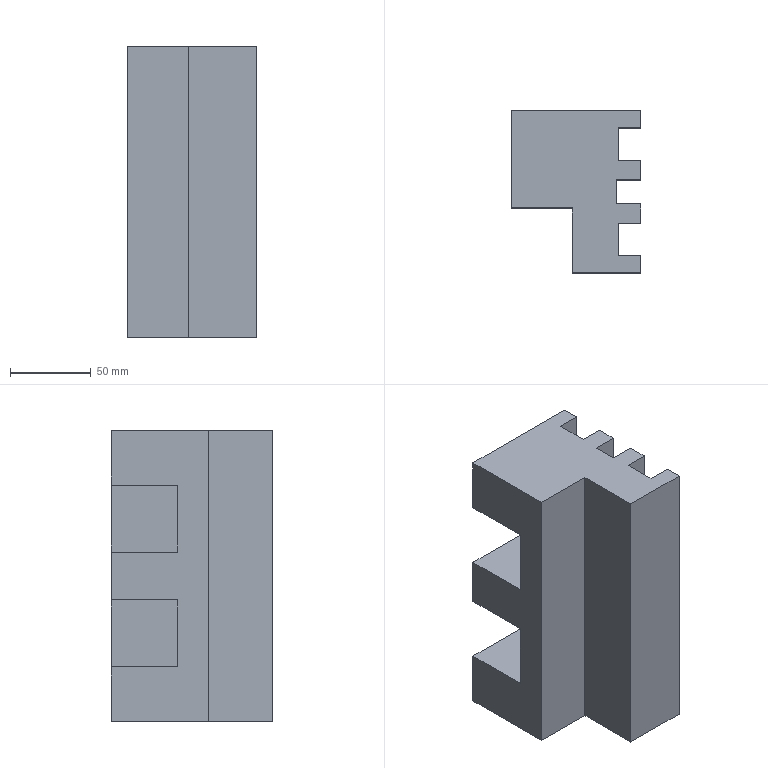Component | SolidWorks | Fixture-2 | 1 solid | 28 faces | box 80 x 100 x 180 mm | volume 866480 mm3 | plane 28
build123d program:
from build123d import *

# Parameters (mm, degrees)
BOSS_EXTRUDE1_DEPTH     = 180
SKETCH2_W               = 46.727
SKETCH2_H               = 41.35
CUT_EXTRUDE1_DEPTH      = 30
CUT_EXTRUDE2_DEPTH      = 221.907
CUT_EXTRUDE2_DEPTH_BACK = 221.907
SKETCH3_W               = 15
SKETCH3_H               = 15
CUT_EXTRUDE3_DEPTH      = 221.907
CUT_EXTRUDE3_DEPTH_BACK = 221.907
SKETCH4_W               = 14
SKETCH4_H               = 20
SKETCH5_W               = 46.727
SKETCH5_H               = 41.35
CUT_EXTRUDE4_DEPTH      = 11.35


with BuildPart() as part:
    # Sketch1 → Boss-Extrude1 (new body)
    with BuildSketch(Plane.XY):
        Polygon((0, 0), (-80, 0), (-80, -60), (-42.162, -60), (-42.162, -100), (0, -100), align=None)
    extrude(amount=BOSS_EXTRUDE1_DEPTH)

    # Sketch2 → Cut-Extrude1 (cut)
    with BuildSketch(Plane(origin=(0, 0, 0), x_dir=(1, 0, 0), z_dir=(0, 1, 0))):
        with Locations((-56.637, -125.435)):
            Rectangle(SKETCH2_W, SKETCH2_H)
        with Locations((-56.637, -54.565)):
            Rectangle(SKETCH2_W, SKETCH2_H)
    extrude(amount=-CUT_EXTRUDE1_DEPTH, mode=Mode.SUBTRACT)

    # Sketch3 → Cut-Extrude2 (cut, two sides: drawn at the far end of the back side and taken through both)
    with BuildSketch(Plane(origin=(0, 0, 0), x_dir=(-1, 0, 0), z_dir=(0, 0, -1)).offset(-CUT_EXTRUDE2_DEPTH_BACK)):
        with Locations((7.5, -50)):
            Rectangle(SKETCH3_W, SKETCH3_H)
    extrude(amount=CUT_EXTRUDE2_DEPTH + CUT_EXTRUDE2_DEPTH_BACK, mode=Mode.SUBTRACT)

    # Sketch4 → Cut-Extrude3 (cut, two sides: drawn at the far end of the back side and taken through both)
    with BuildSketch(Plane(origin=(0, 0, 0), x_dir=(-1, 0, 0), z_dir=(0, 0, -1)).offset(-CUT_EXTRUDE3_DEPTH_BACK)):
        with Locations((7, -20.5)):
            Rectangle(SKETCH4_W, SKETCH4_H)
        with Locations((7, -79.5)):
            Rectangle(SKETCH4_W, SKETCH4_H)
    extrude(amount=CUT_EXTRUDE3_DEPTH + CUT_EXTRUDE3_DEPTH_BACK, mode=Mode.SUBTRACT)

    # Sketch5 → Cut-Extrude4 (cut)
    with BuildSketch(Plane(origin=(0, -30, 0), x_dir=(1, 0, 0), z_dir=(0, 1, 0))):
        with Locations((-56.637, -125.435)):
            Rectangle(SKETCH5_W, SKETCH5_H)
        with Locations((-56.637, -54.565)):
            Rectangle(SKETCH5_W, SKETCH5_H)
    extrude(amount=-CUT_EXTRUDE4_DEPTH, mode=Mode.SUBTRACT)


solid = part.part

# Placed as in the assembly
solid = solid.moved(Location((-136.557, 55.832, -117.351), (0, 0, 0)))
STEP:
#1=COLOUR_RGB('',0.7922,0.8196,0.9333);
#2=FILL_AREA_STYLE_COLOUR('',#1);
#3=FILL_AREA_STYLE('',(#2));
#4=SURFACE_STYLE_FILL_AREA(#3);
#5=SURFACE_SIDE_STYLE('',(#4));
#6=SURFACE_STYLE_USAGE(.BOTH.,#5);
#7=PRESENTATION_STYLE_ASSIGNMENT((#6));
#8=CARTESIAN_POINT('',(-5.376,1.785,2.466));
#9=VERTEX_POINT('',#8);
#10=CARTESIAN_POINT('',(-5.376,2.198,2.466));
#11=VERTEX_POINT('',#10);
#12=CARTESIAN_POINT('',(-5.376,2.198,2.466));
#13=DIRECTION('',(-0.,1.,0.));
#14=VECTOR('',#13,39.37);
#15=LINE('',#12,#14);
#16=EDGE_CURVE('',#9,#11,#15,.T.);
#17=ORIENTED_EDGE('',*,*,#16,.F.);
#18=CARTESIAN_POINT('',(-5.376,1.785,-4.62));
#19=VERTEX_POINT('',#18);
#20=CARTESIAN_POINT('',(-5.376,1.785,2.466));
#21=DIRECTION('',(0.,0.,-1.));
#22=VECTOR('',#21,39.37);
#23=LINE('',#20,#22);
#24=EDGE_CURVE('',#9,#19,#23,.T.);
#25=ORIENTED_EDGE('',*,*,#24,.T.);
#26=CARTESIAN_POINT('',(-5.376,2.198,-4.62));
#27=VERTEX_POINT('',#26);
#28=CARTESIAN_POINT('',(-5.376,2.198,-4.62));
#29=DIRECTION('',(-0.,1.,0.));
#30=VECTOR('',#29,39.37);
#31=LINE('',#28,#30);
#32=EDGE_CURVE('',#19,#27,#31,.T.);
#33=ORIENTED_EDGE('',*,*,#32,.T.);
#34=CARTESIAN_POINT('',(-5.376,2.198,2.466));
#35=DIRECTION('',(0.,0.,-1.));
#36=VECTOR('',#35,39.37);
#37=LINE('',#34,#36);
#38=EDGE_CURVE('',#11,#27,#37,.T.);
#39=ORIENTED_EDGE('',*,*,#38,.F.);
#40=EDGE_LOOP('',(#17,#25,#33,#39));
#41=FACE_OUTER_BOUND('',#40,.T.);
#42=CARTESIAN_POINT('',(-5.376,2.198,2.466));
#43=DIRECTION('',(-1.,-0.,0.));
#44=DIRECTION('',(0.,-1.,0.));
#45=AXIS2_PLACEMENT_3D('',#42,#43,#44);
#46=PLANE('',#45);
#47=ADVANCED_FACE('',(#41),#46,.F.);
#48=CARTESIAN_POINT('',(-5.376,-1.739,-4.62));
#49=VERTEX_POINT('',#48);
#50=CARTESIAN_POINT('',(-5.376,-1.326,-4.62));
#51=VERTEX_POINT('',#50);
#52=CARTESIAN_POINT('',(-5.376,2.198,-4.62));
#53=DIRECTION('',(-0.,1.,0.));
#54=VECTOR('',#53,39.37);
#55=LINE('',#52,#54);
#56=EDGE_CURVE('',#49,#51,#55,.T.);
#57=ORIENTED_EDGE('',*,*,#56,.T.);
#58=CARTESIAN_POINT('',(-5.376,-1.326,2.466));
#59=VERTEX_POINT('',#58);
#60=CARTESIAN_POINT('',(-5.376,-1.326,2.466));
#61=DIRECTION('',(0.,0.,-1.));
#62=VECTOR('',#61,39.37);
#63=LINE('',#60,#62);
#64=EDGE_CURVE('',#59,#51,#63,.T.);
#65=ORIENTED_EDGE('',*,*,#64,.F.);
#66=CARTESIAN_POINT('',(-5.376,-1.739,2.466));
#67=VERTEX_POINT('',#66);
#68=CARTESIAN_POINT('',(-5.376,2.198,2.466));
#69=DIRECTION('',(-0.,1.,0.));
#70=VECTOR('',#69,39.37);
#71=LINE('',#68,#70);
#72=EDGE_CURVE('',#67,#59,#71,.T.);
#73=ORIENTED_EDGE('',*,*,#72,.F.);
#74=CARTESIAN_POINT('',(-5.376,-1.739,2.466));
#75=DIRECTION('',(0.,0.,-1.));
#76=VECTOR('',#75,39.37);
#77=LINE('',#74,#76);
#78=EDGE_CURVE('',#67,#49,#77,.T.);
#79=ORIENTED_EDGE('',*,*,#78,.T.);
#80=EDGE_LOOP('',(#57,#65,#73,#79));
#81=FACE_OUTER_BOUND('',#80,.T.);
#82=CARTESIAN_POINT('',(-5.376,2.198,2.466));
#83=DIRECTION('',(-1.,-0.,0.));
#84=DIRECTION('',(0.,-1.,0.));
#85=AXIS2_PLACEMENT_3D('',#82,#83,#84);
#86=PLANE('',#85);
#87=ADVANCED_FACE('',(#81),#86,.F.);
#88=CARTESIAN_POINT('',(-5.376,0.5249,-4.62));
#89=VERTEX_POINT('',#88);
#90=CARTESIAN_POINT('',(-5.376,0.9973,-4.62));
#91=VERTEX_POINT('',#90);
#92=CARTESIAN_POINT('',(-5.376,2.198,-4.62));
#93=DIRECTION('',(-0.,1.,0.));
#94=VECTOR('',#93,39.37);
#95=LINE('',#92,#94);
#96=EDGE_CURVE('',#89,#91,#95,.T.);
#97=ORIENTED_EDGE('',*,*,#96,.T.);
#98=CARTESIAN_POINT('',(-5.376,0.9973,2.466));
#99=VERTEX_POINT('',#98);
#100=CARTESIAN_POINT('',(-5.376,0.9973,2.466));
#101=DIRECTION('',(0.,0.,-1.));
#102=VECTOR('',#101,39.37);
#103=LINE('',#100,#102);
#104=EDGE_CURVE('',#99,#91,#103,.T.);
#105=ORIENTED_EDGE('',*,*,#104,.F.);
#106=CARTESIAN_POINT('',(-5.376,0.5249,2.466));
#107=VERTEX_POINT('',#106);
#108=CARTESIAN_POINT('',(-5.376,2.198,2.466));
#109=DIRECTION('',(-0.,1.,0.));
#110=VECTOR('',#109,39.37);
#111=LINE('',#108,#110);
#112=EDGE_CURVE('',#107,#99,#111,.T.);
#113=ORIENTED_EDGE('',*,*,#112,.F.);
#114=CARTESIAN_POINT('',(-5.376,0.5249,2.466));
#115=DIRECTION('',(0.,0.,-1.));
#116=VECTOR('',#115,39.37);
#117=LINE('',#114,#116);
#118=EDGE_CURVE('',#107,#89,#117,.T.);
#119=ORIENTED_EDGE('',*,*,#118,.T.);
#120=EDGE_LOOP('',(#97,#105,#113,#119));
#121=FACE_OUTER_BOUND('',#120,.T.);
#122=CARTESIAN_POINT('',(-5.376,2.198,2.466));
#123=DIRECTION('',(-1.,-0.,0.));
#124=DIRECTION('',(0.,-1.,0.));
#125=AXIS2_PLACEMENT_3D('',#122,#123,#124);
#126=PLANE('',#125);
#127=ADVANCED_FACE('',(#121),#126,.F.);
#128=CARTESIAN_POINT('',(-8.526,2.198,-0.4957));
#129=VERTEX_POINT('',#128);
#130=CARTESIAN_POINT('',(-6.686,2.198,-0.4957));
#131=VERTEX_POINT('',#130);
#132=CARTESIAN_POINT('',(-5.376,2.198,-0.4957));
#133=DIRECTION('',(1.,0.,0.));
#134=VECTOR('',#133,39.37);
#135=LINE('',#132,#134);
#136=EDGE_CURVE('',#129,#131,#135,.T.);
#137=ORIENTED_EDGE('',*,*,#136,.T.);
#138=CARTESIAN_POINT('',(-6.686,2.198,1.132));
#139=VERTEX_POINT('',#138);
#140=CARTESIAN_POINT('',(-6.686,2.198,-4.62));
#141=DIRECTION('',(0.,0.,-1.));
#142=VECTOR('',#141,39.37);
#143=LINE('',#140,#142);
#144=EDGE_CURVE('',#139,#131,#143,.T.);
#145=ORIENTED_EDGE('',*,*,#144,.F.);
#146=CARTESIAN_POINT('',(-8.526,2.198,1.132));
#147=VERTEX_POINT('',#146);
#148=CARTESIAN_POINT('',(-5.376,2.198,1.132));
#149=DIRECTION('',(1.,0.,0.));
#150=VECTOR('',#149,39.37);
#151=LINE('',#148,#150);
#152=EDGE_CURVE('',#147,#139,#151,.T.);
#153=ORIENTED_EDGE('',*,*,#152,.F.);
#154=CARTESIAN_POINT('',(-8.526,2.198,2.466));
#155=VERTEX_POINT('',#154);
#156=CARTESIAN_POINT('',(-8.526,2.198,2.466));
#157=DIRECTION('',(0.,0.,-1.));
#158=VECTOR('',#157,39.37);
#159=LINE('',#156,#158);
#160=EDGE_CURVE('',#155,#147,#159,.T.);
#161=ORIENTED_EDGE('',*,*,#160,.F.);
#162=CARTESIAN_POINT('',(-5.376,2.198,2.466));
#163=DIRECTION('',(-1.,-0.,0.));
#164=VECTOR('',#163,39.37);
#165=LINE('',#162,#164);
#166=EDGE_CURVE('',#11,#155,#165,.T.);
#167=ORIENTED_EDGE('',*,*,#166,.F.);
#168=ORIENTED_EDGE('',*,*,#38,.T.);
#169=CARTESIAN_POINT('',(-8.526,2.198,-4.62));
#170=VERTEX_POINT('',#169);
#171=CARTESIAN_POINT('',(-5.376,2.198,-4.62));
#172=DIRECTION('',(-1.,-0.,0.));
#173=VECTOR('',#172,39.37);
#174=LINE('',#171,#173);
#175=EDGE_CURVE('',#27,#170,#174,.T.);
#176=ORIENTED_EDGE('',*,*,#175,.T.);
#177=CARTESIAN_POINT('',(-8.526,2.198,-3.286));
#178=VERTEX_POINT('',#177);
#179=CARTESIAN_POINT('',(-8.526,2.198,2.466));
#180=DIRECTION('',(0.,0.,-1.));
#181=VECTOR('',#180,39.37);
#182=LINE('',#179,#181);
#183=EDGE_CURVE('',#178,#170,#182,.T.);
#184=ORIENTED_EDGE('',*,*,#183,.F.);
#185=CARTESIAN_POINT('',(-6.686,2.198,-3.286));
#186=VERTEX_POINT('',#185);
#187=CARTESIAN_POINT('',(-8.526,2.198,-3.286));
#188=DIRECTION('',(1.,0.,0.));
#189=VECTOR('',#188,39.37);
#190=LINE('',#187,#189);
#191=EDGE_CURVE('',#178,#186,#190,.T.);
#192=ORIENTED_EDGE('',*,*,#191,.T.);
#193=CARTESIAN_POINT('',(-6.686,2.198,-1.658));
#194=VERTEX_POINT('',#193);
#195=CARTESIAN_POINT('',(-6.686,2.198,-3.286));
#196=DIRECTION('',(0.,0.,1.));
#197=VECTOR('',#196,39.37);
#198=LINE('',#195,#197);
#199=EDGE_CURVE('',#186,#194,#198,.T.);
#200=ORIENTED_EDGE('',*,*,#199,.T.);
#201=CARTESIAN_POINT('',(-8.526,2.198,-1.658));
#202=VERTEX_POINT('',#201);
#203=CARTESIAN_POINT('',(-8.526,2.198,-1.658));
#204=DIRECTION('',(1.,0.,0.));
#205=VECTOR('',#204,39.37);
#206=LINE('',#203,#205);
#207=EDGE_CURVE('',#202,#194,#206,.T.);
#208=ORIENTED_EDGE('',*,*,#207,.F.);
#209=CARTESIAN_POINT('',(-8.526,2.198,2.466));
#210=DIRECTION('',(0.,0.,-1.));
#211=VECTOR('',#210,39.37);
#212=LINE('',#209,#211);
#213=EDGE_CURVE('',#129,#202,#212,.T.);
#214=ORIENTED_EDGE('',*,*,#213,.F.);
#215=EDGE_LOOP('',(#137,#145,#153,#161,#167,#168,#176,#184,#192,#200,#208,#214));
#216=FACE_OUTER_BOUND('',#215,.T.);
#217=CARTESIAN_POINT('',(-5.376,2.198,2.466));
#218=DIRECTION('',(0.,-1.,0.));
#219=DIRECTION('',(1.,0.,0.));
#220=AXIS2_PLACEMENT_3D('',#217,#218,#219);
#221=PLANE('',#220);
#222=ADVANCED_FACE('',(#216),#221,.F.);
#223=CARTESIAN_POINT('',(-8.526,0.5701,-0.4957));
#224=VERTEX_POINT('',#223);
#225=CARTESIAN_POINT('',(-8.526,0.5701,1.132));
#226=VERTEX_POINT('',#225);
#227=CARTESIAN_POINT('',(-8.526,0.5701,-0.4957));
#228=DIRECTION('',(-0.,0.,1.));
#229=VECTOR('',#228,39.37);
#230=LINE('',#227,#229);
#231=EDGE_CURVE('',#224,#226,#230,.T.);
#232=ORIENTED_EDGE('',*,*,#231,.F.);
#233=CARTESIAN_POINT('',(-8.526,1.017,-0.4957));
#234=DIRECTION('',(-0.,1.,0.));
#235=VECTOR('',#234,39.37);
#236=LINE('',#233,#235);
#237=EDGE_CURVE('',#224,#129,#236,.T.);
#238=ORIENTED_EDGE('',*,*,#237,.T.);
#239=ORIENTED_EDGE('',*,*,#213,.T.);
#240=CARTESIAN_POINT('',(-8.526,0.5701,-1.658));
#241=VERTEX_POINT('',#240);
#242=CARTESIAN_POINT('',(-8.526,1.017,-1.658));
#243=DIRECTION('',(-0.,1.,0.));
#244=VECTOR('',#243,39.37);
#245=LINE('',#242,#244);
#246=EDGE_CURVE('',#241,#202,#245,.T.);
#247=ORIENTED_EDGE('',*,*,#246,.F.);
#248=CARTESIAN_POINT('',(-8.526,0.5701,-3.286));
#249=VERTEX_POINT('',#248);
#250=CARTESIAN_POINT('',(-8.526,0.5701,-3.286));
#251=DIRECTION('',(-0.,0.,1.));
#252=VECTOR('',#251,39.37);
#253=LINE('',#250,#252);
#254=EDGE_CURVE('',#249,#241,#253,.T.);
#255=ORIENTED_EDGE('',*,*,#254,.F.);
#256=CARTESIAN_POINT('',(-8.526,1.017,-3.286));
#257=DIRECTION('',(-0.,1.,0.));
#258=VECTOR('',#257,39.37);
#259=LINE('',#256,#258);
#260=EDGE_CURVE('',#249,#178,#259,.T.);
#261=ORIENTED_EDGE('',*,*,#260,.T.);
#262=ORIENTED_EDGE('',*,*,#183,.T.);
#263=CARTESIAN_POINT('',(-8.526,-0.1641,-4.62));
#264=VERTEX_POINT('',#263);
#265=CARTESIAN_POINT('',(-8.526,2.198,-4.62));
#266=DIRECTION('',(0.,-1.,0.));
#267=VECTOR('',#266,39.37);
#268=LINE('',#265,#267);
#269=EDGE_CURVE('',#170,#264,#268,.T.);
#270=ORIENTED_EDGE('',*,*,#269,.T.);
#271=CARTESIAN_POINT('',(-8.526,-0.1641,2.466));
#272=VERTEX_POINT('',#271);
#273=CARTESIAN_POINT('',(-8.526,-0.1641,2.466));
#274=DIRECTION('',(0.,0.,-1.));
#275=VECTOR('',#274,39.37);
#276=LINE('',#273,#275);
#277=EDGE_CURVE('',#272,#264,#276,.T.);
#278=ORIENTED_EDGE('',*,*,#277,.F.);
#279=CARTESIAN_POINT('',(-8.526,2.198,2.466));
#280=DIRECTION('',(0.,-1.,0.));
#281=VECTOR('',#280,39.37);
#282=LINE('',#279,#281);
#283=EDGE_CURVE('',#155,#272,#282,.T.);
#284=ORIENTED_EDGE('',*,*,#283,.F.);
#285=ORIENTED_EDGE('',*,*,#160,.T.);
#286=CARTESIAN_POINT('',(-8.526,1.017,1.132));
#287=DIRECTION('',(-0.,1.,0.));
#288=VECTOR('',#287,39.37);
#289=LINE('',#286,#288);
#290=EDGE_CURVE('',#226,#147,#289,.T.);
#291=ORIENTED_EDGE('',*,*,#290,.F.);
#292=EDGE_LOOP('',(#232,#238,#239,#247,#255,#261,#262,#270,#278,#284,#285,#291));
#293=FACE_OUTER_BOUND('',#292,.T.);
#294=CARTESIAN_POINT('',(-8.526,2.198,2.466));
#295=DIRECTION('',(1.,0.,0.));
#296=DIRECTION('',(-0.,1.,0.));
#297=AXIS2_PLACEMENT_3D('',#294,#295,#296);
#298=PLANE('',#297);
#299=ADVANCED_FACE('',(#293),#298,.F.);
#300=CARTESIAN_POINT('',(-5.376,-0.5381,2.466));
#301=VERTEX_POINT('',#300);
#302=CARTESIAN_POINT('',(-5.376,-0.06568,2.466));
#303=VERTEX_POINT('',#302);
#304=CARTESIAN_POINT('',(-5.376,2.198,2.466));
#305=DIRECTION('',(-0.,1.,0.));
#306=VECTOR('',#305,39.37);
#307=LINE('',#304,#306);
#308=EDGE_CURVE('',#301,#303,#307,.T.);
#309=ORIENTED_EDGE('',*,*,#308,.F.);
#310=CARTESIAN_POINT('',(-5.376,-0.5381,-4.62));
#311=VERTEX_POINT('',#310);
#312=CARTESIAN_POINT('',(-5.376,-0.5381,2.466));
#313=DIRECTION('',(0.,0.,-1.));
#314=VECTOR('',#313,39.37);
#315=LINE('',#312,#314);
#316=EDGE_CURVE('',#301,#311,#315,.T.);
#317=ORIENTED_EDGE('',*,*,#316,.T.);
#318=CARTESIAN_POINT('',(-5.376,-0.06568,-4.62));
#319=VERTEX_POINT('',#318);
#320=CARTESIAN_POINT('',(-5.376,2.198,-4.62));
#321=DIRECTION('',(-0.,1.,0.));
#322=VECTOR('',#321,39.37);
#323=LINE('',#320,#322);
#324=EDGE_CURVE('',#311,#319,#323,.T.);
#325=ORIENTED_EDGE('',*,*,#324,.T.);
#326=CARTESIAN_POINT('',(-5.376,-0.06568,2.466));
#327=DIRECTION('',(0.,0.,-1.));
#328=VECTOR('',#327,39.37);
#329=LINE('',#326,#328);
#330=EDGE_CURVE('',#303,#319,#329,.T.);
#331=ORIENTED_EDGE('',*,*,#330,.F.);
#332=EDGE_LOOP('',(#309,#317,#325,#331));
#333=FACE_OUTER_BOUND('',#332,.T.);
#334=CARTESIAN_POINT('',(-5.376,2.198,2.466));
#335=DIRECTION('',(-1.,-0.,0.));
#336=DIRECTION('',(0.,-1.,0.));
#337=AXIS2_PLACEMENT_3D('',#334,#335,#336);
#338=PLANE('',#337);
#339=ADVANCED_FACE('',(#333),#338,.F.);
#340=CARTESIAN_POINT('',(-7.036,-0.1641,-4.62));
#341=VERTEX_POINT('',#340);
#342=CARTESIAN_POINT('',(-7.036,-0.1641,-4.62));
#343=DIRECTION('',(1.,0.,0.));
#344=VECTOR('',#343,39.37);
#345=LINE('',#342,#344);
#346=EDGE_CURVE('',#264,#341,#345,.T.);
#347=ORIENTED_EDGE('',*,*,#346,.T.);
#348=CARTESIAN_POINT('',(-7.036,-0.1641,2.466));
#349=VERTEX_POINT('',#348);
#350=CARTESIAN_POINT('',(-7.036,-0.1641,2.466));
#351=DIRECTION('',(0.,0.,-1.));
#352=VECTOR('',#351,39.37);
#353=LINE('',#350,#352);
#354=EDGE_CURVE('',#349,#341,#353,.T.);
#355=ORIENTED_EDGE('',*,*,#354,.F.);
#356=CARTESIAN_POINT('',(-7.036,-0.1641,2.466));
#357=DIRECTION('',(1.,0.,0.));
#358=VECTOR('',#357,39.37);
#359=LINE('',#356,#358);
#360=EDGE_CURVE('',#272,#349,#359,.T.);
#361=ORIENTED_EDGE('',*,*,#360,.F.);
#362=ORIENTED_EDGE('',*,*,#277,.T.);
#363=EDGE_LOOP('',(#347,#355,#361,#362));
#364=FACE_OUTER_BOUND('',#363,.T.);
#365=CARTESIAN_POINT('',(-7.036,-0.1641,2.466));
#366=DIRECTION('',(-0.,1.,0.));
#367=DIRECTION('',(-1.,-0.,0.));
#368=AXIS2_PLACEMENT_3D('',#365,#366,#367);
#369=PLANE('',#368);
#370=ADVANCED_FACE('',(#364),#369,.F.);
#371=CARTESIAN_POINT('',(-7.036,-1.739,-4.62));
#372=VERTEX_POINT('',#371);
#373=CARTESIAN_POINT('',(-7.036,-1.739,-4.62));
#374=DIRECTION('',(-0.,-1.,0.));
#375=VECTOR('',#374,39.37);
#376=LINE('',#373,#375);
#377=EDGE_CURVE('',#341,#372,#376,.T.);
#378=ORIENTED_EDGE('',*,*,#377,.T.);
#379=CARTESIAN_POINT('',(-7.036,-1.739,2.466));
#380=VERTEX_POINT('',#379);
#381=CARTESIAN_POINT('',(-7.036,-1.739,2.466));
#382=DIRECTION('',(0.,0.,-1.));
#383=VECTOR('',#382,39.37);
#384=LINE('',#381,#383);
#385=EDGE_CURVE('',#380,#372,#384,.T.);
#386=ORIENTED_EDGE('',*,*,#385,.F.);
#387=CARTESIAN_POINT('',(-7.036,-1.739,2.466));
#388=DIRECTION('',(-0.,-1.,0.));
#389=VECTOR('',#388,39.37);
#390=LINE('',#387,#389);
#391=EDGE_CURVE('',#349,#380,#390,.T.);
#392=ORIENTED_EDGE('',*,*,#391,.F.);
#393=ORIENTED_EDGE('',*,*,#354,.T.);
#394=EDGE_LOOP('',(#378,#386,#392,#393));
#395=FACE_OUTER_BOUND('',#394,.T.);
#396=CARTESIAN_POINT('',(-7.036,-1.739,2.466));
#397=DIRECTION('',(1.,-0.,0.));
#398=DIRECTION('',(0.,1.,0.));
#399=AXIS2_PLACEMENT_3D('',#396,#397,#398);
#400=PLANE('',#399);
#401=ADVANCED_FACE('',(#395),#400,.F.);
#402=CARTESIAN_POINT('',(-5.376,-1.739,-4.62));
#403=DIRECTION('',(1.,0.,0.));
#404=VECTOR('',#403,39.37);
#405=LINE('',#402,#404);
#406=EDGE_CURVE('',#372,#49,#405,.T.);
#407=ORIENTED_EDGE('',*,*,#406,.T.);
#408=ORIENTED_EDGE('',*,*,#78,.F.);
#409=CARTESIAN_POINT('',(-5.376,-1.739,2.466));
#410=DIRECTION('',(1.,0.,0.));
#411=VECTOR('',#410,39.37);
#412=LINE('',#409,#411);
#413=EDGE_CURVE('',#380,#67,#412,.T.);
#414=ORIENTED_EDGE('',*,*,#413,.F.);
#415=ORIENTED_EDGE('',*,*,#385,.T.);
#416=EDGE_LOOP('',(#407,#408,#414,#415));
#417=FACE_OUTER_BOUND('',#416,.T.);
#418=CARTESIAN_POINT('',(-5.376,-1.739,2.466));
#419=DIRECTION('',(0.,1.,0.));
#420=DIRECTION('',(0.,0.,1.));
#421=AXIS2_PLACEMENT_3D('',#418,#419,#420);
#422=PLANE('',#421);
#423=ADVANCED_FACE('',(#417),#422,.F.);
#424=CARTESIAN_POINT('',(-5.927,0.9973,2.466));
#425=VERTEX_POINT('',#424);
#426=CARTESIAN_POINT('',(-5.927,1.785,2.466));
#427=VERTEX_POINT('',#426);
#428=CARTESIAN_POINT('',(-5.927,1.785,2.466));
#429=DIRECTION('',(0.,1.,0.));
#430=VECTOR('',#429,39.37);
#431=LINE('',#428,#430);
#432=EDGE_CURVE('',#425,#427,#431,.T.);
#433=ORIENTED_EDGE('',*,*,#432,.T.);
#434=CARTESIAN_POINT('',(-5.376,1.785,2.466));
#435=DIRECTION('',(1.,0.,0.));
#436=VECTOR('',#435,39.37);
#437=LINE('',#434,#436);
#438=EDGE_CURVE('',#427,#9,#437,.T.);
#439=ORIENTED_EDGE('',*,*,#438,.T.);
#440=ORIENTED_EDGE('',*,*,#16,.T.);
#441=ORIENTED_EDGE('',*,*,#166,.T.);
#442=ORIENTED_EDGE('',*,*,#283,.T.);
#443=ORIENTED_EDGE('',*,*,#360,.T.);
#444=ORIENTED_EDGE('',*,*,#391,.T.);
#445=ORIENTED_EDGE('',*,*,#413,.T.);
#446=ORIENTED_EDGE('',*,*,#72,.T.);
#447=CARTESIAN_POINT('',(-5.927,-1.326,2.466));
#448=VERTEX_POINT('',#447);
#449=CARTESIAN_POINT('',(-5.376,-1.326,2.466));
#450=DIRECTION('',(-1.,0.,0.));
#451=VECTOR('',#450,39.37);
#452=LINE('',#449,#451);
#453=EDGE_CURVE('',#59,#448,#452,.T.);
#454=ORIENTED_EDGE('',*,*,#453,.T.);
#455=CARTESIAN_POINT('',(-5.927,-0.5381,2.466));
#456=VERTEX_POINT('',#455);
#457=CARTESIAN_POINT('',(-5.927,-1.326,2.466));
#458=DIRECTION('',(-0.,1.,0.));
#459=VECTOR('',#458,39.37);
#460=LINE('',#457,#459);
#461=EDGE_CURVE('',#448,#456,#460,.T.);
#462=ORIENTED_EDGE('',*,*,#461,.T.);
#463=CARTESIAN_POINT('',(-5.376,-0.5381,2.466));
#464=DIRECTION('',(1.,0.,0.));
#465=VECTOR('',#464,39.37);
#466=LINE('',#463,#465);
#467=EDGE_CURVE('',#456,#301,#466,.T.);
#468=ORIENTED_EDGE('',*,*,#467,.T.);
#469=ORIENTED_EDGE('',*,*,#308,.T.);
#470=CARTESIAN_POINT('',(-5.967,-0.06568,2.466));
#471=VERTEX_POINT('',#470);
#472=CARTESIAN_POINT('',(-5.376,-0.06568,2.466));
#473=DIRECTION('',(-1.,0.,0.));
#474=VECTOR('',#473,39.37);
#475=LINE('',#472,#474);
#476=EDGE_CURVE('',#303,#471,#475,.T.);
#477=ORIENTED_EDGE('',*,*,#476,.T.);
#478=CARTESIAN_POINT('',(-5.967,0.5249,2.466));
#479=VERTEX_POINT('',#478);
#480=CARTESIAN_POINT('',(-5.967,0.5249,2.466));
#481=DIRECTION('',(0.,1.,0.));
#482=VECTOR('',#481,39.37);
#483=LINE('',#480,#482);
#484=EDGE_CURVE('',#471,#479,#483,.T.);
#485=ORIENTED_EDGE('',*,*,#484,.T.);
#486=CARTESIAN_POINT('',(-5.376,0.5249,2.466));
#487=DIRECTION('',(1.,0.,0.));
#488=VECTOR('',#487,39.37);
#489=LINE('',#486,#488);
#490=EDGE_CURVE('',#479,#107,#489,.T.);
#491=ORIENTED_EDGE('',*,*,#490,.T.);
#492=ORIENTED_EDGE('',*,*,#112,.T.);
#493=CARTESIAN_POINT('',(-5.376,0.9973,2.466));
#494=DIRECTION('',(-1.,0.,0.));
#495=VECTOR('',#494,39.37);
#496=LINE('',#493,#495);
#497=EDGE_CURVE('',#99,#425,#496,.T.);
#498=ORIENTED_EDGE('',*,*,#497,.T.);
#499=EDGE_LOOP('',(#433,#439,#440,#441,#442,#443,#444,#445,#446,#454,#462,#468,#469,#477,#485,#491,#492,#498));
#500=FACE_OUTER_BOUND('',#499,.T.);
#501=CARTESIAN_POINT('',(-5.376,2.198,2.466));
#502=DIRECTION('',(0.,0.,-1.));
#503=DIRECTION('',(-1.,0.,0.));
#504=AXIS2_PLACEMENT_3D('',#501,#502,#503);
#505=PLANE('',#504);
#506=ADVANCED_FACE('',(#500),#505,.F.);
#507=CARTESIAN_POINT('',(-5.927,1.785,-4.62));
#508=VERTEX_POINT('',#507);
#509=CARTESIAN_POINT('',(-5.376,1.785,-4.62));
#510=DIRECTION('',(1.,0.,0.));
#511=VECTOR('',#510,39.37);
#512=LINE('',#509,#511);
#513=EDGE_CURVE('',#508,#19,#512,.T.);
#514=ORIENTED_EDGE('',*,*,#513,.F.);
#515=CARTESIAN_POINT('',(-5.927,0.9973,-4.62));
#516=VERTEX_POINT('',#515);
#517=CARTESIAN_POINT('',(-5.927,2.198,-4.62));
#518=DIRECTION('',(0.,1.,0.));
#519=VECTOR('',#518,39.37);
#520=LINE('',#517,#519);
#521=EDGE_CURVE('',#516,#508,#520,.T.);
#522=ORIENTED_EDGE('',*,*,#521,.F.);
#523=CARTESIAN_POINT('',(-5.376,0.9973,-4.62));
#524=DIRECTION('',(-1.,0.,0.));
#525=VECTOR('',#524,39.37);
#526=LINE('',#523,#525);
#527=EDGE_CURVE('',#91,#516,#526,.T.);
#528=ORIENTED_EDGE('',*,*,#527,.F.);
#529=ORIENTED_EDGE('',*,*,#96,.F.);
#530=CARTESIAN_POINT('',(-5.967,0.5249,-4.62));
#531=VERTEX_POINT('',#530);
#532=CARTESIAN_POINT('',(-5.376,0.5249,-4.62));
#533=DIRECTION('',(1.,0.,0.));
#534=VECTOR('',#533,39.37);
#535=LINE('',#532,#534);
#536=EDGE_CURVE('',#531,#89,#535,.T.);
#537=ORIENTED_EDGE('',*,*,#536,.F.);
#538=CARTESIAN_POINT('',(-5.967,-0.06568,-4.62));
#539=VERTEX_POINT('',#538);
#540=CARTESIAN_POINT('',(-5.967,2.198,-4.62));
#541=DIRECTION('',(0.,1.,0.));
#542=VECTOR('',#541,39.37);
#543=LINE('',#540,#542);
#544=EDGE_CURVE('',#539,#531,#543,.T.);
#545=ORIENTED_EDGE('',*,*,#544,.F.);
#546=CARTESIAN_POINT('',(-5.376,-0.06568,-4.62));
#547=DIRECTION('',(-1.,0.,0.));
#548=VECTOR('',#547,39.37);
#549=LINE('',#546,#548);
#550=EDGE_CURVE('',#319,#539,#549,.T.);
#551=ORIENTED_EDGE('',*,*,#550,.F.);
#552=ORIENTED_EDGE('',*,*,#324,.F.);
#553=CARTESIAN_POINT('',(-5.927,-0.5381,-4.62));
#554=VERTEX_POINT('',#553);
#555=CARTESIAN_POINT('',(-5.376,-0.5381,-4.62));
#556=DIRECTION('',(1.,0.,0.));
#557=VECTOR('',#556,39.37);
#558=LINE('',#555,#557);
#559=EDGE_CURVE('',#554,#311,#558,.T.);
#560=ORIENTED_EDGE('',*,*,#559,.F.);
#561=CARTESIAN_POINT('',(-5.927,-1.326,-4.62));
#562=VERTEX_POINT('',#561);
#563=CARTESIAN_POINT('',(-5.927,2.198,-4.62));
#564=DIRECTION('',(-0.,1.,0.));
#565=VECTOR('',#564,39.37);
#566=LINE('',#563,#565);
#567=EDGE_CURVE('',#562,#554,#566,.T.);
#568=ORIENTED_EDGE('',*,*,#567,.F.);
#569=CARTESIAN_POINT('',(-5.376,-1.326,-4.62));
#570=DIRECTION('',(-1.,0.,0.));
#571=VECTOR('',#570,39.37);
#572=LINE('',#569,#571);
#573=EDGE_CURVE('',#51,#562,#572,.T.);
#574=ORIENTED_EDGE('',*,*,#573,.F.);
#575=ORIENTED_EDGE('',*,*,#56,.F.);
#576=ORIENTED_EDGE('',*,*,#406,.F.);
#577=ORIENTED_EDGE('',*,*,#377,.F.);
#578=ORIENTED_EDGE('',*,*,#346,.F.);
#579=ORIENTED_EDGE('',*,*,#269,.F.);
#580=ORIENTED_EDGE('',*,*,#175,.F.);
#581=ORIENTED_EDGE('',*,*,#32,.F.);
#582=EDGE_LOOP('',(#514,#522,#528,#529,#537,#545,#551,#552,#560,#568,#574,#575,#576,#577,#578,#579,#580,#581));
#583=FACE_OUTER_BOUND('',#582,.T.);
#584=CARTESIAN_POINT('',(-5.376,2.198,-4.62));
#585=DIRECTION('',(0.,0.,-1.));
#586=DIRECTION('',(-1.,0.,0.));
#587=AXIS2_PLACEMENT_3D('',#584,#585,#586);
#588=PLANE('',#587);
#589=ADVANCED_FACE('',(#583),#588,.T.);
#590=ORIENTED_EDGE('',*,*,#207,.T.);
#591=CARTESIAN_POINT('',(-6.686,0.5701,-1.658));
#592=VERTEX_POINT('',#591);
#593=CARTESIAN_POINT('',(-6.686,1.017,-1.658));
#594=DIRECTION('',(-0.,1.,0.));
#595=VECTOR('',#594,39.37);
#596=LINE('',#593,#595);
#597=EDGE_CURVE('',#592,#194,#596,.T.);
#598=ORIENTED_EDGE('',*,*,#597,.F.);
#599=CARTESIAN_POINT('',(-8.526,0.5701,-1.658));
#600=DIRECTION('',(1.,0.,0.));
#601=VECTOR('',#600,39.37);
#602=LINE('',#599,#601);
#603=EDGE_CURVE('',#241,#592,#602,.T.);
#604=ORIENTED_EDGE('',*,*,#603,.F.);
#605=ORIENTED_EDGE('',*,*,#246,.T.);
#606=EDGE_LOOP('',(#590,#598,#604,#605));
#607=FACE_OUTER_BOUND('',#606,.T.);
#608=CARTESIAN_POINT('',(-8.526,1.017,-1.658));
#609=DIRECTION('',(0.,0.,1.));
#610=DIRECTION('',(1.,0.,0.));
#611=AXIS2_PLACEMENT_3D('',#608,#609,#610);
#612=PLANE('',#611);
#613=ADVANCED_FACE('',(#607),#612,.F.);
#614=ORIENTED_EDGE('',*,*,#191,.F.);
#615=ORIENTED_EDGE('',*,*,#260,.F.);
#616=CARTESIAN_POINT('',(-6.686,0.5701,-3.286));
#617=VERTEX_POINT('',#616);
#618=CARTESIAN_POINT('',(-6.686,0.5701,-3.286));
#619=DIRECTION('',(-1.,-0.,0.));
#620=VECTOR('',#619,39.37);
#621=LINE('',#618,#620);
#622=EDGE_CURVE('',#617,#249,#621,.T.);
#623=ORIENTED_EDGE('',*,*,#622,.F.);
#624=CARTESIAN_POINT('',(-6.686,1.017,-3.286));
#625=DIRECTION('',(-0.,1.,0.));
#626=VECTOR('',#625,39.37);
#627=LINE('',#624,#626);
#628=EDGE_CURVE('',#617,#186,#627,.T.);
#629=ORIENTED_EDGE('',*,*,#628,.T.);
#630=EDGE_LOOP('',(#614,#615,#623,#629));
#631=FACE_OUTER_BOUND('',#630,.T.);
#632=CARTESIAN_POINT('',(-8.526,1.017,-3.286));
#633=DIRECTION('',(0.,0.,1.));
#634=DIRECTION('',(1.,0.,0.));
#635=AXIS2_PLACEMENT_3D('',#632,#633,#634);
#636=PLANE('',#635);
#637=ADVANCED_FACE('',(#631),#636,.T.);
#638=ORIENTED_EDGE('',*,*,#199,.F.);
#639=ORIENTED_EDGE('',*,*,#628,.F.);
#640=CARTESIAN_POINT('',(-6.686,0.5701,-1.658));
#641=DIRECTION('',(-0.,0.,-1.));
#642=VECTOR('',#641,39.37);
#643=LINE('',#640,#642);
#644=EDGE_CURVE('',#592,#617,#643,.T.);
#645=ORIENTED_EDGE('',*,*,#644,.F.);
#646=ORIENTED_EDGE('',*,*,#597,.T.);
#647=EDGE_LOOP('',(#638,#639,#645,#646));
#648=FACE_OUTER_BOUND('',#647,.T.);
#649=CARTESIAN_POINT('',(-6.686,1.017,-3.286));
#650=DIRECTION('',(-1.,-0.,0.));
#651=DIRECTION('',(0.,0.,1.));
#652=AXIS2_PLACEMENT_3D('',#649,#650,#651);
#653=PLANE('',#652);
#654=ADVANCED_FACE('',(#648),#653,.T.);
#655=ORIENTED_EDGE('',*,*,#136,.F.);
#656=ORIENTED_EDGE('',*,*,#237,.F.);
#657=CARTESIAN_POINT('',(-6.686,0.5701,-0.4957));
#658=VERTEX_POINT('',#657);
#659=CARTESIAN_POINT('',(-6.686,0.5701,-0.4957));
#660=DIRECTION('',(-1.,-0.,0.));
#661=VECTOR('',#660,39.37);
#662=LINE('',#659,#661);
#663=EDGE_CURVE('',#658,#224,#662,.T.);
#664=ORIENTED_EDGE('',*,*,#663,.F.);
#665=CARTESIAN_POINT('',(-6.686,1.017,-0.4957));
#666=DIRECTION('',(-0.,1.,0.));
#667=VECTOR('',#666,39.37);
#668=LINE('',#665,#667);
#669=EDGE_CURVE('',#658,#131,#668,.T.);
#670=ORIENTED_EDGE('',*,*,#669,.T.);
#671=EDGE_LOOP('',(#655,#656,#664,#670));
#672=FACE_OUTER_BOUND('',#671,.T.);
#673=CARTESIAN_POINT('',(-5.376,1.017,-0.4957));
#674=DIRECTION('',(0.,0.,1.));
#675=DIRECTION('',(1.,0.,0.));
#676=AXIS2_PLACEMENT_3D('',#673,#674,#675);
#677=PLANE('',#676);
#678=ADVANCED_FACE('',(#672),#677,.T.);
#679=ORIENTED_EDGE('',*,*,#144,.T.);
#680=ORIENTED_EDGE('',*,*,#669,.F.);
#681=CARTESIAN_POINT('',(-6.686,0.5701,1.132));
#682=VERTEX_POINT('',#681);
#683=CARTESIAN_POINT('',(-6.686,0.5701,1.132));
#684=DIRECTION('',(0.,0.,-1.));
#685=VECTOR('',#684,39.37);
#686=LINE('',#683,#685);
#687=EDGE_CURVE('',#682,#658,#686,.T.);
#688=ORIENTED_EDGE('',*,*,#687,.F.);
#689=CARTESIAN_POINT('',(-6.686,1.017,1.132));
#690=DIRECTION('',(-0.,1.,0.));
#691=VECTOR('',#690,39.37);
#692=LINE('',#689,#691);
#693=EDGE_CURVE('',#682,#139,#692,.T.);
#694=ORIENTED_EDGE('',*,*,#693,.T.);
#695=EDGE_LOOP('',(#679,#680,#688,#694));
#696=FACE_OUTER_BOUND('',#695,.T.);
#697=CARTESIAN_POINT('',(-6.686,1.017,-4.62));
#698=DIRECTION('',(1.,0.,0.));
#699=DIRECTION('',(0.,0.,-1.));
#700=AXIS2_PLACEMENT_3D('',#697,#698,#699);
#701=PLANE('',#700);
#702=ADVANCED_FACE('',(#696),#701,.F.);
#703=ORIENTED_EDGE('',*,*,#152,.T.);
#704=ORIENTED_EDGE('',*,*,#693,.F.);
#705=CARTESIAN_POINT('',(-8.526,0.5701,1.132));
#706=DIRECTION('',(1.,0.,0.));
#707=VECTOR('',#706,39.37);
#708=LINE('',#705,#707);
#709=EDGE_CURVE('',#226,#682,#708,.T.);
#710=ORIENTED_EDGE('',*,*,#709,.F.);
#711=ORIENTED_EDGE('',*,*,#290,.T.);
#712=EDGE_LOOP('',(#703,#704,#710,#711));
#713=FACE_OUTER_BOUND('',#712,.T.);
#714=CARTESIAN_POINT('',(-5.376,1.017,1.132));
#715=DIRECTION('',(0.,0.,1.));
#716=DIRECTION('',(1.,0.,0.));
#717=AXIS2_PLACEMENT_3D('',#714,#715,#716);
#718=PLANE('',#717);
#719=ADVANCED_FACE('',(#713),#718,.F.);
#720=ORIENTED_EDGE('',*,*,#536,.T.);
#721=ORIENTED_EDGE('',*,*,#118,.F.);
#722=ORIENTED_EDGE('',*,*,#490,.F.);
#723=CARTESIAN_POINT('',(-5.967,0.5249,2.466));
#724=DIRECTION('',(0.,0.,-1.));
#725=VECTOR('',#724,39.37);
#726=LINE('',#723,#725);
#727=EDGE_CURVE('',#479,#531,#726,.T.);
#728=ORIENTED_EDGE('',*,*,#727,.T.);
#729=EDGE_LOOP('',(#720,#721,#722,#728));
#730=FACE_OUTER_BOUND('',#729,.T.);
#731=CARTESIAN_POINT('',(-5.376,0.5249,2.466));
#732=DIRECTION('',(0.,1.,0.));
#733=DIRECTION('',(0.,0.,1.));
#734=AXIS2_PLACEMENT_3D('',#731,#732,#733);
#735=PLANE('',#734);
#736=ADVANCED_FACE('',(#730),#735,.F.);
#737=ORIENTED_EDGE('',*,*,#544,.T.);
#738=ORIENTED_EDGE('',*,*,#727,.F.);
#739=ORIENTED_EDGE('',*,*,#484,.F.);
#740=CARTESIAN_POINT('',(-5.967,-0.06568,2.466));
#741=DIRECTION('',(0.,0.,-1.));
#742=VECTOR('',#741,39.37);
#743=LINE('',#740,#742);
#744=EDGE_CURVE('',#471,#539,#743,.T.);
#745=ORIENTED_EDGE('',*,*,#744,.T.);
#746=EDGE_LOOP('',(#737,#738,#739,#745));
#747=FACE_OUTER_BOUND('',#746,.T.);
#748=CARTESIAN_POINT('',(-5.967,0.5249,2.466));
#749=DIRECTION('',(-1.,0.,0.));
#750=DIRECTION('',(-0.,-1.,0.));
#751=AXIS2_PLACEMENT_3D('',#748,#749,#750);
#752=PLANE('',#751);
#753=ADVANCED_FACE('',(#747),#752,.F.);
#754=ORIENTED_EDGE('',*,*,#550,.T.);
#755=ORIENTED_EDGE('',*,*,#744,.F.);
#756=ORIENTED_EDGE('',*,*,#476,.F.);
#757=ORIENTED_EDGE('',*,*,#330,.T.);
#758=EDGE_LOOP('',(#754,#755,#756,#757));
#759=FACE_OUTER_BOUND('',#758,.T.);
#760=CARTESIAN_POINT('',(-5.376,-0.06568,2.466));
#761=DIRECTION('',(0.,-1.,0.));
#762=DIRECTION('',(0.,0.,-1.));
#763=AXIS2_PLACEMENT_3D('',#760,#761,#762);
#764=PLANE('',#763);
#765=ADVANCED_FACE('',(#759),#764,.F.);
#766=ORIENTED_EDGE('',*,*,#573,.T.);
#767=CARTESIAN_POINT('',(-5.927,-1.326,2.466));
#768=DIRECTION('',(0.,0.,-1.));
#769=VECTOR('',#768,39.37);
#770=LINE('',#767,#769);
#771=EDGE_CURVE('',#448,#562,#770,.T.);
#772=ORIENTED_EDGE('',*,*,#771,.F.);
#773=ORIENTED_EDGE('',*,*,#453,.F.);
#774=ORIENTED_EDGE('',*,*,#64,.T.);
#775=EDGE_LOOP('',(#766,#772,#773,#774));
#776=FACE_OUTER_BOUND('',#775,.T.);
#777=CARTESIAN_POINT('',(-5.376,-1.326,2.466));
#778=DIRECTION('',(0.,-1.,0.));
#779=DIRECTION('',(0.,0.,-1.));
#780=AXIS2_PLACEMENT_3D('',#777,#778,#779);
#781=PLANE('',#780);
#782=ADVANCED_FACE('',(#776),#781,.F.);
#783=ORIENTED_EDGE('',*,*,#559,.T.);
#784=ORIENTED_EDGE('',*,*,#316,.F.);
#785=ORIENTED_EDGE('',*,*,#467,.F.);
#786=CARTESIAN_POINT('',(-5.927,-0.5381,2.466));
#787=DIRECTION('',(0.,0.,-1.));
#788=VECTOR('',#787,39.37);
#789=LINE('',#786,#788);
#790=EDGE_CURVE('',#456,#554,#789,.T.);
#791=ORIENTED_EDGE('',*,*,#790,.T.);
#792=EDGE_LOOP('',(#783,#784,#785,#791));
#793=FACE_OUTER_BOUND('',#792,.T.);
#794=CARTESIAN_POINT('',(-5.376,-0.5381,2.466));
#795=DIRECTION('',(0.,1.,0.));
#796=DIRECTION('',(0.,0.,1.));
#797=AXIS2_PLACEMENT_3D('',#794,#795,#796);
#798=PLANE('',#797);
#799=ADVANCED_FACE('',(#793),#798,.F.);
#800=ORIENTED_EDGE('',*,*,#567,.T.);
#801=ORIENTED_EDGE('',*,*,#790,.F.);
#802=ORIENTED_EDGE('',*,*,#461,.F.);
#803=ORIENTED_EDGE('',*,*,#771,.T.);
#804=EDGE_LOOP('',(#800,#801,#802,#803));
#805=FACE_OUTER_BOUND('',#804,.T.);
#806=CARTESIAN_POINT('',(-5.927,-1.326,2.466));
#807=DIRECTION('',(-1.,-0.,0.));
#808=DIRECTION('',(0.,-1.,0.));
#809=AXIS2_PLACEMENT_3D('',#806,#807,#808);
#810=PLANE('',#809);
#811=ADVANCED_FACE('',(#805),#810,.F.);
#812=ORIENTED_EDGE('',*,*,#513,.T.);
#813=ORIENTED_EDGE('',*,*,#24,.F.);
#814=ORIENTED_EDGE('',*,*,#438,.F.);
#815=CARTESIAN_POINT('',(-5.927,1.785,2.466));
#816=DIRECTION('',(0.,0.,-1.));
#817=VECTOR('',#816,39.37);
#818=LINE('',#815,#817);
#819=EDGE_CURVE('',#427,#508,#818,.T.);
#820=ORIENTED_EDGE('',*,*,#819,.T.);
#821=EDGE_LOOP('',(#812,#813,#814,#820));
#822=FACE_OUTER_BOUND('',#821,.T.);
#823=CARTESIAN_POINT('',(-5.376,1.785,2.466));
#824=DIRECTION('',(0.,1.,0.));
#825=DIRECTION('',(0.,0.,1.));
#826=AXIS2_PLACEMENT_3D('',#823,#824,#825);
#827=PLANE('',#826);
#828=ADVANCED_FACE('',(#822),#827,.F.);
#829=ORIENTED_EDGE('',*,*,#521,.T.);
#830=ORIENTED_EDGE('',*,*,#819,.F.);
#831=ORIENTED_EDGE('',*,*,#432,.F.);
#832=CARTESIAN_POINT('',(-5.927,0.9973,2.466));
#833=DIRECTION('',(0.,0.,-1.));
#834=VECTOR('',#833,39.37);
#835=LINE('',#832,#834);
#836=EDGE_CURVE('',#425,#516,#835,.T.);
#837=ORIENTED_EDGE('',*,*,#836,.T.);
#838=EDGE_LOOP('',(#829,#830,#831,#837));
#839=FACE_OUTER_BOUND('',#838,.T.);
#840=CARTESIAN_POINT('',(-5.927,1.785,2.466));
#841=DIRECTION('',(-1.,0.,0.));
#842=DIRECTION('',(-0.,-1.,0.));
#843=AXIS2_PLACEMENT_3D('',#840,#841,#842);
#844=PLANE('',#843);
#845=ADVANCED_FACE('',(#839),#844,.F.);
#846=ORIENTED_EDGE('',*,*,#527,.T.);
#847=ORIENTED_EDGE('',*,*,#836,.F.);
#848=ORIENTED_EDGE('',*,*,#497,.F.);
#849=ORIENTED_EDGE('',*,*,#104,.T.);
#850=EDGE_LOOP('',(#846,#847,#848,#849));
#851=FACE_OUTER_BOUND('',#850,.T.);
#852=CARTESIAN_POINT('',(-5.376,0.9973,2.466));
#853=DIRECTION('',(0.,-1.,0.));
#854=DIRECTION('',(0.,0.,-1.));
#855=AXIS2_PLACEMENT_3D('',#852,#853,#854);
#856=PLANE('',#855);
#857=ADVANCED_FACE('',(#851),#856,.F.);
#858=ORIENTED_EDGE('',*,*,#663,.T.);
#859=ORIENTED_EDGE('',*,*,#231,.T.);
#860=ORIENTED_EDGE('',*,*,#709,.T.);
#861=ORIENTED_EDGE('',*,*,#687,.T.);
#862=EDGE_LOOP('',(#858,#859,#860,#861));
#863=FACE_OUTER_BOUND('',#862,.T.);
#864=CARTESIAN_POINT('',(-5.376,0.5701,-4.62));
#865=DIRECTION('',(-0.,1.,-0.));
#866=DIRECTION('',(-1.,-0.,0.));
#867=AXIS2_PLACEMENT_3D('',#864,#865,#866);
#868=PLANE('',#867);
#869=ADVANCED_FACE('',(#863),#868,.T.);
#870=ORIENTED_EDGE('',*,*,#254,.T.);
#871=ORIENTED_EDGE('',*,*,#603,.T.);
#872=ORIENTED_EDGE('',*,*,#644,.T.);
#873=ORIENTED_EDGE('',*,*,#622,.T.);
#874=EDGE_LOOP('',(#870,#871,#872,#873));
#875=FACE_OUTER_BOUND('',#874,.T.);
#876=CARTESIAN_POINT('',(-5.376,0.5701,-4.62));
#877=DIRECTION('',(-0.,1.,-0.));
#878=DIRECTION('',(-1.,-0.,0.));
#879=AXIS2_PLACEMENT_3D('',#876,#877,#878);
#880=PLANE('',#879);
#881=ADVANCED_FACE('',(#875),#880,.T.);
#882=CLOSED_SHELL('',(#47,#87,#127,#222,#299,#339,#370,#401,#423,#506,#589,#613,#637,#654,#678,#702,#719,#736,#753,#765,#782,#799,#811,#828,#845,#857,#869,#881));
#883=MANIFOLD_SOLID_BREP('',#882);
#884=STYLED_ITEM('',(#7),#883);
#885=(LENGTH_UNIT()NAMED_UNIT(*)SI_UNIT($,.METRE.));
#886=LENGTH_MEASURE_WITH_UNIT(LENGTH_MEASURE(0.0254),#885);
#887=DIMENSIONAL_EXPONENTS(1.,0.,0.,0.,0.,0.,0.);
#888=(CONVERSION_BASED_UNIT('',#886)LENGTH_UNIT()NAMED_UNIT(#887));
#889=UNCERTAINTY_MEASURE_WITH_UNIT(LENGTH_MEASURE(0.00001),#888,'','');
#890=(NAMED_UNIT(*)PLANE_ANGLE_UNIT()SI_UNIT($,.RADIAN.));
#891=(NAMED_UNIT(*)SI_UNIT($,.STERADIAN.)SOLID_ANGLE_UNIT());
#892=(GEOMETRIC_REPRESENTATION_CONTEXT(3)GLOBAL_UNCERTAINTY_ASSIGNED_CONTEXT((#889))GLOBAL_UNIT_ASSIGNED_CONTEXT((#888,#890,#891))REPRESENTATION_CONTEXT('',''));
#893=MECHANICAL_DESIGN_GEOMETRIC_PRESENTATION_REPRESENTATION('',(#884),#892);
#894=PRESENTATION_LAYER_ASSIGNMENT('','',(#884));
#895=CARTESIAN_POINT('',(0.,0.,0.));
#896=DIRECTION('',(0.,0.,1.));
#897=DIRECTION('',(1.,0.,0.));
#898=AXIS2_PLACEMENT_3D('',#895,#896,#897);
#899=(LENGTH_UNIT()NAMED_UNIT(*)SI_UNIT($,.METRE.));
#900=LENGTH_MEASURE_WITH_UNIT(LENGTH_MEASURE(0.0254),#899);
#901=DIMENSIONAL_EXPONENTS(1.,0.,0.,0.,0.,0.,0.);
#902=(CONVERSION_BASED_UNIT('',#900)LENGTH_UNIT()NAMED_UNIT(#901));
#903=UNCERTAINTY_MEASURE_WITH_UNIT(LENGTH_MEASURE(0.00001),#902,'','');
#904=(NAMED_UNIT(*)PLANE_ANGLE_UNIT()SI_UNIT($,.RADIAN.));
#905=(NAMED_UNIT(*)SI_UNIT($,.STERADIAN.)SOLID_ANGLE_UNIT());
#906=(GEOMETRIC_REPRESENTATION_CONTEXT(3)GLOBAL_UNCERTAINTY_ASSIGNED_CONTEXT((#903))GLOBAL_UNIT_ASSIGNED_CONTEXT((#902,#904,#905))REPRESENTATION_CONTEXT('',''));
#907=ADVANCED_BREP_SHAPE_REPRESENTATION('',(#883,#898),#906);